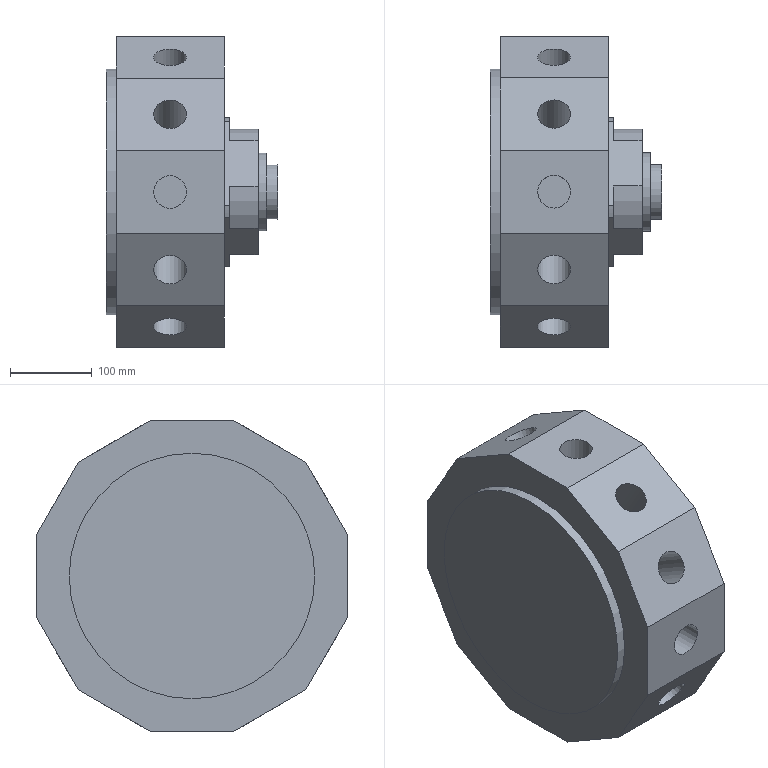Component | NX | SIM15_REV_SCHEIBE | 1 solid | 63 faces | volume 15342647 mm3 | plane 39 | cylinder 23 | cone 1 | commonest cylinder face diameters 40 x12 184 x4 154 x4 300 x1 96 x1 67 x1